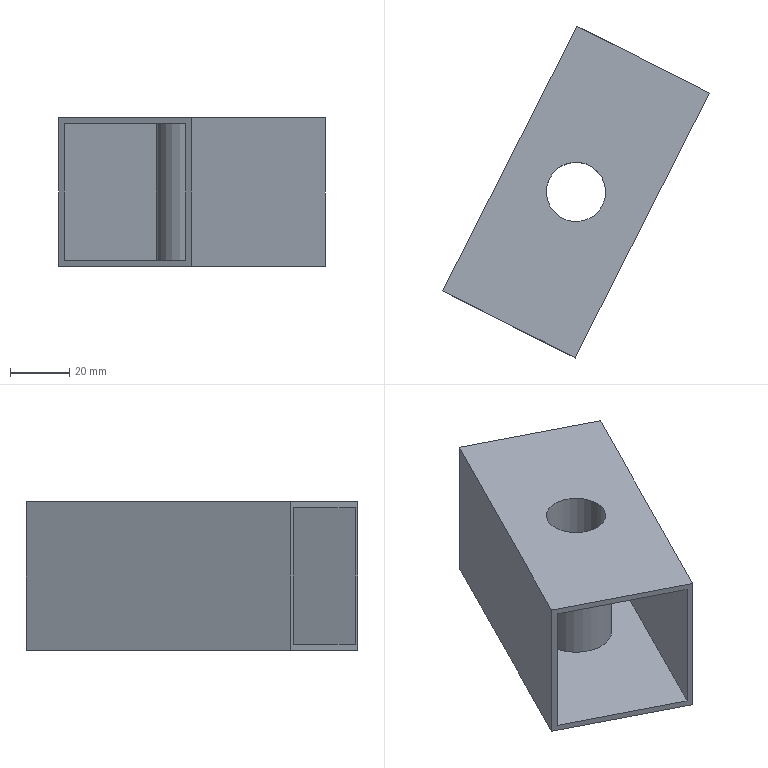Component | SolidWorks | Part28-3 | 1 solid | 14 faces | box 89.81 x 111.8 x 50 mm | volume 43502 mm3 | plane 10 | cylinder 4 | commonest cylinder face diameters 24 x2 20 x2
build123d program:
from build123d import *

# Parameters (mm, degrees)
SKETCH1_W           = 50
SKETCH1_H           = 100
SKETCH1_R           = 10
BOSS_EXTRUDE1_DEPTH = 50
SHELL1_T            = -2


with BuildPart() as part:
    # Sketch1 → Boss-Extrude1 (new body)
    with BuildSketch(Plane.XY):
        with Locations((-21.791, -15.019)):
            Rectangle(SKETCH1_W, SKETCH1_H)
        with Locations((-21.791, -15.019)):
            Circle(SKETCH1_R, mode=Mode.SUBTRACT)
    extrude(amount=BOSS_EXTRUDE1_DEPTH)

    # Shell1
    shell1_openings = [part.faces().sort_by_distance(p)[0] for p in [
        (-21.791, 34.981, 25),
        (-21.791, -65.019, 25),
    ]]
    offset(amount=SHELL1_T, openings=shell1_openings, kind=Kind.INTERSECTION)


solid = part.part

# Placed as in the assembly
solid = solid.moved(Location((-642.419, -825.467, 2539.971), (0, 0, 153.121)))
STEP:
#1=COLOUR_RGB('',0.7922,0.8196,0.9333);
#2=FILL_AREA_STYLE_COLOUR('',#1);
#3=FILL_AREA_STYLE('',(#2));
#4=SURFACE_STYLE_FILL_AREA(#3);
#5=SURFACE_SIDE_STYLE('',(#4));
#6=SURFACE_STYLE_USAGE(.BOTH.,#5);
#7=PRESENTATION_STYLE_ASSIGNMENT((#6));
#8=CARTESIAN_POINT('',(-23.838,-32.573,101.889));
#9=VERTEX_POINT('',#8);
#10=CARTESIAN_POINT('',(-24.681,-32.146,101.889));
#11=VERTEX_POINT('',#10);
#12=CARTESIAN_POINT('',(-24.26,-32.359,101.889));
#13=DIRECTION('',(-0.,-0.,1.));
#14=DIRECTION('',(0.892,-0.4521,-0.));
#15=AXIS2_PLACEMENT_3D('',#12,#13,#14);
#16=CIRCLE('',#15,0.4724);
#17=EDGE_CURVE('',#9,#11,#16,.T.);
#18=ORIENTED_EDGE('',*,*,#17,.F.);
#19=CARTESIAN_POINT('',(-23.838,-32.573,100.078));
#20=VERTEX_POINT('',#19);
#21=CARTESIAN_POINT('',(-23.838,-32.573,101.967));
#22=DIRECTION('',(0.,0.,-1.));
#23=VECTOR('',#22,39.37);
#24=LINE('',#21,#23);
#25=EDGE_CURVE('',#9,#20,#24,.T.);
#26=ORIENTED_EDGE('',*,*,#25,.T.);
#27=CARTESIAN_POINT('',(-24.681,-32.146,100.078));
#28=VERTEX_POINT('',#27);
#29=CARTESIAN_POINT('',(-24.26,-32.359,100.078));
#30=DIRECTION('',(-0.,-0.,1.));
#31=DIRECTION('',(0.892,-0.4521,-0.));
#32=AXIS2_PLACEMENT_3D('',#29,#30,#31);
#33=CIRCLE('',#32,0.4724);
#34=EDGE_CURVE('',#20,#28,#33,.T.);
#35=ORIENTED_EDGE('',*,*,#34,.T.);
#36=CARTESIAN_POINT('',(-24.681,-32.146,101.967));
#37=DIRECTION('',(0.,0.,-1.));
#38=VECTOR('',#37,39.37);
#39=LINE('',#36,#38);
#40=EDGE_CURVE('',#11,#28,#39,.T.);
#41=ORIENTED_EDGE('',*,*,#40,.F.);
#42=EDGE_LOOP('',(#18,#26,#35,#41));
#43=FACE_OUTER_BOUND('',#42,.T.);
#44=CARTESIAN_POINT('',(-24.26,-32.359,101.967));
#45=DIRECTION('',(0.,0.,-1.));
#46=DIRECTION('',(-0.892,0.4521,0.));
#47=AXIS2_PLACEMENT_3D('',#44,#45,#46);
#48=CYLINDRICAL_SURFACE('',#47,0.4724);
#49=ADVANCED_FACE('',(#43),#48,.T.);
#50=CARTESIAN_POINT('',(-24.611,-32.181,101.967));
#51=VERTEX_POINT('',#50);
#52=CARTESIAN_POINT('',(-23.908,-32.537,101.967));
#53=VERTEX_POINT('',#52);
#54=CARTESIAN_POINT('',(-24.26,-32.359,101.967));
#55=DIRECTION('',(-0.,-0.,1.));
#56=DIRECTION('',(0.892,-0.4521,-0.));
#57=AXIS2_PLACEMENT_3D('',#54,#55,#56);
#58=CIRCLE('',#57,0.3937);
#59=EDGE_CURVE('',#51,#53,#58,.T.);
#60=ORIENTED_EDGE('',*,*,#59,.T.);
#61=CARTESIAN_POINT('',(-23.908,-32.537,99.999));
#62=VERTEX_POINT('',#61);
#63=CARTESIAN_POINT('',(-23.908,-32.537,101.967));
#64=DIRECTION('',(0.,0.,-1.));
#65=VECTOR('',#64,39.37);
#66=LINE('',#63,#65);
#67=EDGE_CURVE('',#53,#62,#66,.T.);
#68=ORIENTED_EDGE('',*,*,#67,.T.);
#69=CARTESIAN_POINT('',(-24.611,-32.181,99.999));
#70=VERTEX_POINT('',#69);
#71=CARTESIAN_POINT('',(-24.26,-32.359,99.999));
#72=DIRECTION('',(-0.,-0.,1.));
#73=DIRECTION('',(0.892,-0.4521,-0.));
#74=AXIS2_PLACEMENT_3D('',#71,#72,#73);
#75=CIRCLE('',#74,0.3937);
#76=EDGE_CURVE('',#70,#62,#75,.T.);
#77=ORIENTED_EDGE('',*,*,#76,.F.);
#78=CARTESIAN_POINT('',(-24.611,-32.181,101.967));
#79=DIRECTION('',(0.,0.,-1.));
#80=VECTOR('',#79,39.37);
#81=LINE('',#78,#80);
#82=EDGE_CURVE('',#51,#70,#81,.T.);
#83=ORIENTED_EDGE('',*,*,#82,.F.);
#84=EDGE_LOOP('',(#60,#68,#77,#83));
#85=FACE_OUTER_BOUND('',#84,.T.);
#86=CARTESIAN_POINT('',(-24.26,-32.359,101.967));
#87=DIRECTION('',(0.,0.,-1.));
#88=DIRECTION('',(-0.892,0.4521,0.));
#89=AXIS2_PLACEMENT_3D('',#86,#87,#88);
#90=CYLINDRICAL_SURFACE('',#89,0.3937);
#91=ADVANCED_FACE('',(#85),#90,.F.);
#92=CARTESIAN_POINT('',(-26.027,-33.67,99.999));
#93=VERTEX_POINT('',#92);
#94=CARTESIAN_POINT('',(-24.272,-34.56,99.999));
#95=VERTEX_POINT('',#94);
#96=CARTESIAN_POINT('',(-26.027,-33.67,99.999));
#97=DIRECTION('',(0.892,-0.4521,-0.));
#98=VECTOR('',#97,39.37);
#99=LINE('',#96,#98);
#100=EDGE_CURVE('',#93,#95,#99,.T.);
#101=ORIENTED_EDGE('',*,*,#100,.T.);
#102=CARTESIAN_POINT('',(-24.272,-34.56,101.967));
#103=VERTEX_POINT('',#102);
#104=CARTESIAN_POINT('',(-24.272,-34.56,101.967));
#105=DIRECTION('',(0.,0.,-1.));
#106=VECTOR('',#105,39.37);
#107=LINE('',#104,#106);
#108=EDGE_CURVE('',#103,#95,#107,.T.);
#109=ORIENTED_EDGE('',*,*,#108,.F.);
#110=CARTESIAN_POINT('',(-26.027,-33.67,101.967));
#111=VERTEX_POINT('',#110);
#112=CARTESIAN_POINT('',(-26.027,-33.67,101.967));
#113=DIRECTION('',(0.892,-0.4521,-0.));
#114=VECTOR('',#113,39.37);
#115=LINE('',#112,#114);
#116=EDGE_CURVE('',#111,#103,#115,.T.);
#117=ORIENTED_EDGE('',*,*,#116,.F.);
#118=CARTESIAN_POINT('',(-26.027,-33.67,101.967));
#119=DIRECTION('',(0.,0.,-1.));
#120=VECTOR('',#119,39.37);
#121=LINE('',#118,#120);
#122=EDGE_CURVE('',#111,#93,#121,.T.);
#123=ORIENTED_EDGE('',*,*,#122,.T.);
#124=EDGE_LOOP('',(#101,#109,#117,#123));
#125=FACE_OUTER_BOUND('',#124,.T.);
#126=CARTESIAN_POINT('',(-25.957,-33.706,100.078));
#127=VERTEX_POINT('',#126);
#128=CARTESIAN_POINT('',(-24.342,-34.524,100.078));
#129=VERTEX_POINT('',#128);
#130=CARTESIAN_POINT('',(-26.027,-33.67,100.078));
#131=DIRECTION('',(0.892,-0.4521,-0.));
#132=VECTOR('',#131,39.37);
#133=LINE('',#130,#132);
#134=EDGE_CURVE('',#127,#129,#133,.T.);
#135=ORIENTED_EDGE('',*,*,#134,.F.);
#136=CARTESIAN_POINT('',(-25.957,-33.706,101.889));
#137=VERTEX_POINT('',#136);
#138=CARTESIAN_POINT('',(-25.957,-33.706,101.967));
#139=DIRECTION('',(0.,0.,-1.));
#140=VECTOR('',#139,39.37);
#141=LINE('',#138,#140);
#142=EDGE_CURVE('',#137,#127,#141,.T.);
#143=ORIENTED_EDGE('',*,*,#142,.F.);
#144=CARTESIAN_POINT('',(-24.342,-34.524,101.889));
#145=VERTEX_POINT('',#144);
#146=CARTESIAN_POINT('',(-26.027,-33.67,101.889));
#147=DIRECTION('',(0.892,-0.4521,-0.));
#148=VECTOR('',#147,39.37);
#149=LINE('',#146,#148);
#150=EDGE_CURVE('',#137,#145,#149,.T.);
#151=ORIENTED_EDGE('',*,*,#150,.T.);
#152=CARTESIAN_POINT('',(-24.342,-34.524,101.967));
#153=DIRECTION('',(0.,0.,-1.));
#154=VECTOR('',#153,39.37);
#155=LINE('',#152,#154);
#156=EDGE_CURVE('',#145,#129,#155,.T.);
#157=ORIENTED_EDGE('',*,*,#156,.T.);
#158=EDGE_LOOP('',(#135,#143,#151,#157));
#159=FACE_BOUND('',#158,.T.);
#160=CARTESIAN_POINT('',(-26.027,-33.67,101.967));
#161=DIRECTION('',(0.4521,0.892,0.));
#162=DIRECTION('',(-0.,-0.,1.));
#163=AXIS2_PLACEMENT_3D('',#160,#161,#162);
#164=PLANE('',#163);
#165=ADVANCED_FACE('',(#125,#159),#164,.F.);
#166=CARTESIAN_POINT('',(-22.492,-31.048,99.999));
#167=VERTEX_POINT('',#166);
#168=CARTESIAN_POINT('',(-24.247,-30.158,99.999));
#169=VERTEX_POINT('',#168);
#170=CARTESIAN_POINT('',(-24.247,-30.158,99.999));
#171=DIRECTION('',(-0.892,0.4521,0.));
#172=VECTOR('',#171,39.37);
#173=LINE('',#170,#172);
#174=EDGE_CURVE('',#167,#169,#173,.T.);
#175=ORIENTED_EDGE('',*,*,#174,.T.);
#176=CARTESIAN_POINT('',(-24.247,-30.158,101.967));
#177=VERTEX_POINT('',#176);
#178=CARTESIAN_POINT('',(-24.247,-30.158,101.967));
#179=DIRECTION('',(0.,0.,-1.));
#180=VECTOR('',#179,39.37);
#181=LINE('',#178,#180);
#182=EDGE_CURVE('',#177,#169,#181,.T.);
#183=ORIENTED_EDGE('',*,*,#182,.F.);
#184=CARTESIAN_POINT('',(-22.492,-31.048,101.967));
#185=VERTEX_POINT('',#184);
#186=CARTESIAN_POINT('',(-24.247,-30.158,101.967));
#187=DIRECTION('',(-0.892,0.4521,0.));
#188=VECTOR('',#187,39.37);
#189=LINE('',#186,#188);
#190=EDGE_CURVE('',#185,#177,#189,.T.);
#191=ORIENTED_EDGE('',*,*,#190,.F.);
#192=CARTESIAN_POINT('',(-22.492,-31.048,101.967));
#193=DIRECTION('',(0.,0.,-1.));
#194=VECTOR('',#193,39.37);
#195=LINE('',#192,#194);
#196=EDGE_CURVE('',#185,#167,#195,.T.);
#197=ORIENTED_EDGE('',*,*,#196,.T.);
#198=EDGE_LOOP('',(#175,#183,#191,#197));
#199=FACE_OUTER_BOUND('',#198,.T.);
#200=CARTESIAN_POINT('',(-22.562,-31.013,100.078));
#201=VERTEX_POINT('',#200);
#202=CARTESIAN_POINT('',(-24.177,-30.194,100.078));
#203=VERTEX_POINT('',#202);
#204=CARTESIAN_POINT('',(-24.247,-30.158,100.078));
#205=DIRECTION('',(-0.892,0.4521,0.));
#206=VECTOR('',#205,39.37);
#207=LINE('',#204,#206);
#208=EDGE_CURVE('',#201,#203,#207,.T.);
#209=ORIENTED_EDGE('',*,*,#208,.F.);
#210=CARTESIAN_POINT('',(-22.562,-31.013,101.889));
#211=VERTEX_POINT('',#210);
#212=CARTESIAN_POINT('',(-22.562,-31.013,101.967));
#213=DIRECTION('',(0.,0.,-1.));
#214=VECTOR('',#213,39.37);
#215=LINE('',#212,#214);
#216=EDGE_CURVE('',#211,#201,#215,.T.);
#217=ORIENTED_EDGE('',*,*,#216,.F.);
#218=CARTESIAN_POINT('',(-24.177,-30.194,101.889));
#219=VERTEX_POINT('',#218);
#220=CARTESIAN_POINT('',(-24.247,-30.158,101.889));
#221=DIRECTION('',(-0.892,0.4521,0.));
#222=VECTOR('',#221,39.37);
#223=LINE('',#220,#222);
#224=EDGE_CURVE('',#211,#219,#223,.T.);
#225=ORIENTED_EDGE('',*,*,#224,.T.);
#226=CARTESIAN_POINT('',(-24.177,-30.194,101.967));
#227=DIRECTION('',(0.,0.,-1.));
#228=VECTOR('',#227,39.37);
#229=LINE('',#226,#228);
#230=EDGE_CURVE('',#219,#203,#229,.T.);
#231=ORIENTED_EDGE('',*,*,#230,.T.);
#232=EDGE_LOOP('',(#209,#217,#225,#231));
#233=FACE_BOUND('',#232,.T.);
#234=CARTESIAN_POINT('',(-24.247,-30.158,101.967));
#235=DIRECTION('',(-0.4521,-0.892,-0.));
#236=DIRECTION('',(0.,0.,-1.));
#237=AXIS2_PLACEMENT_3D('',#234,#235,#236);
#238=PLANE('',#237);
#239=ADVANCED_FACE('',(#199,#233),#238,.F.);
#240=CARTESIAN_POINT('',(-24.247,-30.158,101.967));
#241=DIRECTION('',(-0.4521,-0.892,-0.));
#242=VECTOR('',#241,39.37);
#243=LINE('',#240,#242);
#244=EDGE_CURVE('',#177,#111,#243,.T.);
#245=ORIENTED_EDGE('',*,*,#244,.T.);
#246=ORIENTED_EDGE('',*,*,#116,.T.);
#247=CARTESIAN_POINT('',(-22.492,-31.048,101.967));
#248=DIRECTION('',(0.4521,0.892,0.));
#249=VECTOR('',#248,39.37);
#250=LINE('',#247,#249);
#251=EDGE_CURVE('',#103,#185,#250,.T.);
#252=ORIENTED_EDGE('',*,*,#251,.T.);
#253=ORIENTED_EDGE('',*,*,#190,.T.);
#254=EDGE_LOOP('',(#245,#246,#252,#253));
#255=FACE_OUTER_BOUND('',#254,.T.);
#256=ORIENTED_EDGE('',*,*,#59,.F.);
#257=CARTESIAN_POINT('',(-24.26,-32.359,101.967));
#258=DIRECTION('',(-0.,-0.,1.));
#259=DIRECTION('',(0.892,-0.4521,-0.));
#260=AXIS2_PLACEMENT_3D('',#257,#258,#259);
#261=CIRCLE('',#260,0.3937);
#262=EDGE_CURVE('',#53,#51,#261,.T.);
#263=ORIENTED_EDGE('',*,*,#262,.F.);
#264=EDGE_LOOP('',(#256,#263));
#265=FACE_BOUND('',#264,.T.);
#266=CARTESIAN_POINT('',(-23.227,-32.22,101.967));
#267=DIRECTION('',(-0.,-0.,1.));
#268=DIRECTION('',(0.892,-0.4521,-0.));
#269=AXIS2_PLACEMENT_3D('',#266,#267,#268);
#270=PLANE('',#269);
#271=ADVANCED_FACE('',(#255,#265),#270,.T.);
#272=CARTESIAN_POINT('',(-24.247,-30.158,99.999));
#273=DIRECTION('',(-0.4521,-0.892,-0.));
#274=VECTOR('',#273,39.37);
#275=LINE('',#272,#274);
#276=EDGE_CURVE('',#169,#93,#275,.T.);
#277=ORIENTED_EDGE('',*,*,#276,.F.);
#278=ORIENTED_EDGE('',*,*,#174,.F.);
#279=CARTESIAN_POINT('',(-22.492,-31.048,99.999));
#280=DIRECTION('',(0.4521,0.892,0.));
#281=VECTOR('',#280,39.37);
#282=LINE('',#279,#281);
#283=EDGE_CURVE('',#95,#167,#282,.T.);
#284=ORIENTED_EDGE('',*,*,#283,.F.);
#285=ORIENTED_EDGE('',*,*,#100,.F.);
#286=EDGE_LOOP('',(#277,#278,#284,#285));
#287=FACE_OUTER_BOUND('',#286,.T.);
#288=ORIENTED_EDGE('',*,*,#76,.T.);
#289=CARTESIAN_POINT('',(-24.26,-32.359,99.999));
#290=DIRECTION('',(-0.,-0.,1.));
#291=DIRECTION('',(0.892,-0.4521,-0.));
#292=AXIS2_PLACEMENT_3D('',#289,#290,#291);
#293=CIRCLE('',#292,0.3937);
#294=EDGE_CURVE('',#62,#70,#293,.T.);
#295=ORIENTED_EDGE('',*,*,#294,.T.);
#296=EDGE_LOOP('',(#288,#295));
#297=FACE_BOUND('',#296,.T.);
#298=CARTESIAN_POINT('',(-23.227,-32.22,99.999));
#299=DIRECTION('',(-0.,-0.,1.));
#300=DIRECTION('',(0.892,-0.4521,-0.));
#301=AXIS2_PLACEMENT_3D('',#298,#299,#300);
#302=PLANE('',#301);
#303=ADVANCED_FACE('',(#287,#297),#302,.F.);
#304=ORIENTED_EDGE('',*,*,#276,.T.);
#305=ORIENTED_EDGE('',*,*,#122,.F.);
#306=ORIENTED_EDGE('',*,*,#244,.F.);
#307=ORIENTED_EDGE('',*,*,#182,.T.);
#308=EDGE_LOOP('',(#304,#305,#306,#307));
#309=FACE_OUTER_BOUND('',#308,.T.);
#310=CARTESIAN_POINT('',(-24.247,-30.158,101.967));
#311=DIRECTION('',(0.892,-0.4521,-0.));
#312=DIRECTION('',(0.4521,0.892,0.));
#313=AXIS2_PLACEMENT_3D('',#310,#311,#312);
#314=PLANE('',#313);
#315=ADVANCED_FACE('',(#309),#314,.F.);
#316=ORIENTED_EDGE('',*,*,#283,.T.);
#317=ORIENTED_EDGE('',*,*,#196,.F.);
#318=ORIENTED_EDGE('',*,*,#251,.F.);
#319=ORIENTED_EDGE('',*,*,#108,.T.);
#320=EDGE_LOOP('',(#316,#317,#318,#319));
#321=FACE_OUTER_BOUND('',#320,.T.);
#322=CARTESIAN_POINT('',(-22.492,-31.048,101.967));
#323=DIRECTION('',(-0.892,0.4521,0.));
#324=DIRECTION('',(-0.4521,-0.892,-0.));
#325=AXIS2_PLACEMENT_3D('',#322,#323,#324);
#326=PLANE('',#325);
#327=ADVANCED_FACE('',(#321),#326,.F.);
#328=ORIENTED_EDGE('',*,*,#67,.F.);
#329=ORIENTED_EDGE('',*,*,#262,.T.);
#330=ORIENTED_EDGE('',*,*,#82,.T.);
#331=ORIENTED_EDGE('',*,*,#294,.F.);
#332=EDGE_LOOP('',(#328,#329,#330,#331));
#333=FACE_OUTER_BOUND('',#332,.T.);
#334=CARTESIAN_POINT('',(-24.26,-32.359,101.967));
#335=DIRECTION('',(0.,0.,-1.));
#336=DIRECTION('',(-0.892,0.4521,0.));
#337=AXIS2_PLACEMENT_3D('',#334,#335,#336);
#338=CYLINDRICAL_SURFACE('',#337,0.3937);
#339=ADVANCED_FACE('',(#333),#338,.F.);
#340=CARTESIAN_POINT('',(-24.177,-30.194,101.889));
#341=DIRECTION('',(-0.4521,-0.892,-0.));
#342=VECTOR('',#341,39.37);
#343=LINE('',#340,#342);
#344=EDGE_CURVE('',#219,#137,#343,.T.);
#345=ORIENTED_EDGE('',*,*,#344,.F.);
#346=ORIENTED_EDGE('',*,*,#224,.F.);
#347=CARTESIAN_POINT('',(-22.562,-31.013,101.889));
#348=DIRECTION('',(0.4521,0.892,0.));
#349=VECTOR('',#348,39.37);
#350=LINE('',#347,#349);
#351=EDGE_CURVE('',#145,#211,#350,.T.);
#352=ORIENTED_EDGE('',*,*,#351,.F.);
#353=ORIENTED_EDGE('',*,*,#150,.F.);
#354=EDGE_LOOP('',(#345,#346,#352,#353));
#355=FACE_OUTER_BOUND('',#354,.T.);
#356=CARTESIAN_POINT('',(-24.26,-32.359,101.889));
#357=DIRECTION('',(-0.,-0.,1.));
#358=DIRECTION('',(0.892,-0.4521,-0.));
#359=AXIS2_PLACEMENT_3D('',#356,#357,#358);
#360=CIRCLE('',#359,0.4724);
#361=EDGE_CURVE('',#11,#9,#360,.T.);
#362=ORIENTED_EDGE('',*,*,#361,.T.);
#363=ORIENTED_EDGE('',*,*,#17,.T.);
#364=EDGE_LOOP('',(#362,#363));
#365=FACE_BOUND('',#364,.T.);
#366=CARTESIAN_POINT('',(-23.227,-32.22,101.889));
#367=DIRECTION('',(-0.,-0.,1.));
#368=DIRECTION('',(0.892,-0.4521,-0.));
#369=AXIS2_PLACEMENT_3D('',#366,#367,#368);
#370=PLANE('',#369);
#371=ADVANCED_FACE('',(#355,#365),#370,.F.);
#372=CARTESIAN_POINT('',(-24.177,-30.194,100.078));
#373=DIRECTION('',(-0.4521,-0.892,-0.));
#374=VECTOR('',#373,39.37);
#375=LINE('',#372,#374);
#376=EDGE_CURVE('',#203,#127,#375,.T.);
#377=ORIENTED_EDGE('',*,*,#376,.T.);
#378=ORIENTED_EDGE('',*,*,#134,.T.);
#379=CARTESIAN_POINT('',(-22.562,-31.013,100.078));
#380=DIRECTION('',(0.4521,0.892,0.));
#381=VECTOR('',#380,39.37);
#382=LINE('',#379,#381);
#383=EDGE_CURVE('',#129,#201,#382,.T.);
#384=ORIENTED_EDGE('',*,*,#383,.T.);
#385=ORIENTED_EDGE('',*,*,#208,.T.);
#386=EDGE_LOOP('',(#377,#378,#384,#385));
#387=FACE_OUTER_BOUND('',#386,.T.);
#388=CARTESIAN_POINT('',(-24.26,-32.359,100.078));
#389=DIRECTION('',(-0.,-0.,1.));
#390=DIRECTION('',(0.892,-0.4521,-0.));
#391=AXIS2_PLACEMENT_3D('',#388,#389,#390);
#392=CIRCLE('',#391,0.4724);
#393=EDGE_CURVE('',#28,#20,#392,.T.);
#394=ORIENTED_EDGE('',*,*,#393,.F.);
#395=ORIENTED_EDGE('',*,*,#34,.F.);
#396=EDGE_LOOP('',(#394,#395));
#397=FACE_BOUND('',#396,.T.);
#398=CARTESIAN_POINT('',(-23.227,-32.22,100.078));
#399=DIRECTION('',(-0.,-0.,1.));
#400=DIRECTION('',(0.892,-0.4521,-0.));
#401=AXIS2_PLACEMENT_3D('',#398,#399,#400);
#402=PLANE('',#401);
#403=ADVANCED_FACE('',(#387,#397),#402,.T.);
#404=ORIENTED_EDGE('',*,*,#376,.F.);
#405=ORIENTED_EDGE('',*,*,#230,.F.);
#406=ORIENTED_EDGE('',*,*,#344,.T.);
#407=ORIENTED_EDGE('',*,*,#142,.T.);
#408=EDGE_LOOP('',(#404,#405,#406,#407));
#409=FACE_OUTER_BOUND('',#408,.T.);
#410=CARTESIAN_POINT('',(-24.177,-30.194,101.967));
#411=DIRECTION('',(0.892,-0.4521,-0.));
#412=DIRECTION('',(0.4521,0.892,0.));
#413=AXIS2_PLACEMENT_3D('',#410,#411,#412);
#414=PLANE('',#413);
#415=ADVANCED_FACE('',(#409),#414,.T.);
#416=ORIENTED_EDGE('',*,*,#383,.F.);
#417=ORIENTED_EDGE('',*,*,#156,.F.);
#418=ORIENTED_EDGE('',*,*,#351,.T.);
#419=ORIENTED_EDGE('',*,*,#216,.T.);
#420=EDGE_LOOP('',(#416,#417,#418,#419));
#421=FACE_OUTER_BOUND('',#420,.T.);
#422=CARTESIAN_POINT('',(-22.562,-31.013,101.967));
#423=DIRECTION('',(-0.892,0.4521,0.));
#424=DIRECTION('',(-0.4521,-0.892,-0.));
#425=AXIS2_PLACEMENT_3D('',#422,#423,#424);
#426=PLANE('',#425);
#427=ADVANCED_FACE('',(#421),#426,.T.);
#428=ORIENTED_EDGE('',*,*,#25,.F.);
#429=ORIENTED_EDGE('',*,*,#361,.F.);
#430=ORIENTED_EDGE('',*,*,#40,.T.);
#431=ORIENTED_EDGE('',*,*,#393,.T.);
#432=EDGE_LOOP('',(#428,#429,#430,#431));
#433=FACE_OUTER_BOUND('',#432,.T.);
#434=CARTESIAN_POINT('',(-24.26,-32.359,101.967));
#435=DIRECTION('',(0.,0.,-1.));
#436=DIRECTION('',(-0.892,0.4521,0.));
#437=AXIS2_PLACEMENT_3D('',#434,#435,#436);
#438=CYLINDRICAL_SURFACE('',#437,0.4724);
#439=ADVANCED_FACE('',(#433),#438,.T.);
#440=CLOSED_SHELL('',(#49,#91,#165,#239,#271,#303,#315,#327,#339,#371,#403,#415,#427,#439));
#441=MANIFOLD_SOLID_BREP('',#440);
#442=STYLED_ITEM('',(#7),#441);
#443=(LENGTH_UNIT()NAMED_UNIT(*)SI_UNIT($,.METRE.));
#444=LENGTH_MEASURE_WITH_UNIT(LENGTH_MEASURE(0.0254),#443);
#445=DIMENSIONAL_EXPONENTS(1.,0.,0.,0.,0.,0.,0.);
#446=(CONVERSION_BASED_UNIT('',#444)LENGTH_UNIT()NAMED_UNIT(#445));
#447=UNCERTAINTY_MEASURE_WITH_UNIT(LENGTH_MEASURE(0.00001),#446,'','');
#448=(NAMED_UNIT(*)PLANE_ANGLE_UNIT()SI_UNIT($,.RADIAN.));
#449=(NAMED_UNIT(*)SI_UNIT($,.STERADIAN.)SOLID_ANGLE_UNIT());
#450=(GEOMETRIC_REPRESENTATION_CONTEXT(3)GLOBAL_UNCERTAINTY_ASSIGNED_CONTEXT((#447))GLOBAL_UNIT_ASSIGNED_CONTEXT((#446,#448,#449))REPRESENTATION_CONTEXT('',''));
#451=MECHANICAL_DESIGN_GEOMETRIC_PRESENTATION_REPRESENTATION('',(#442),#450);
#452=CARTESIAN_POINT('',(0.,0.,0.));
#453=DIRECTION('',(0.,0.,1.));
#454=DIRECTION('',(1.,0.,0.));
#455=AXIS2_PLACEMENT_3D('',#452,#453,#454);
#456=(LENGTH_UNIT()NAMED_UNIT(*)SI_UNIT($,.METRE.));
#457=LENGTH_MEASURE_WITH_UNIT(LENGTH_MEASURE(0.0254),#456);
#458=DIMENSIONAL_EXPONENTS(1.,0.,0.,0.,0.,0.,0.);
#459=(CONVERSION_BASED_UNIT('',#457)LENGTH_UNIT()NAMED_UNIT(#458));
#460=UNCERTAINTY_MEASURE_WITH_UNIT(LENGTH_MEASURE(0.00001),#459,'','');
#461=(NAMED_UNIT(*)PLANE_ANGLE_UNIT()SI_UNIT($,.RADIAN.));
#462=(NAMED_UNIT(*)SI_UNIT($,.STERADIAN.)SOLID_ANGLE_UNIT());
#463=(GEOMETRIC_REPRESENTATION_CONTEXT(3)GLOBAL_UNCERTAINTY_ASSIGNED_CONTEXT((#460))GLOBAL_UNIT_ASSIGNED_CONTEXT((#459,#461,#462))REPRESENTATION_CONTEXT('',''));
#464=ADVANCED_BREP_SHAPE_REPRESENTATION('',(#441,#455),#463);
#465=PRESENTATION_LAYER_ASSIGNMENT('','',(#442));